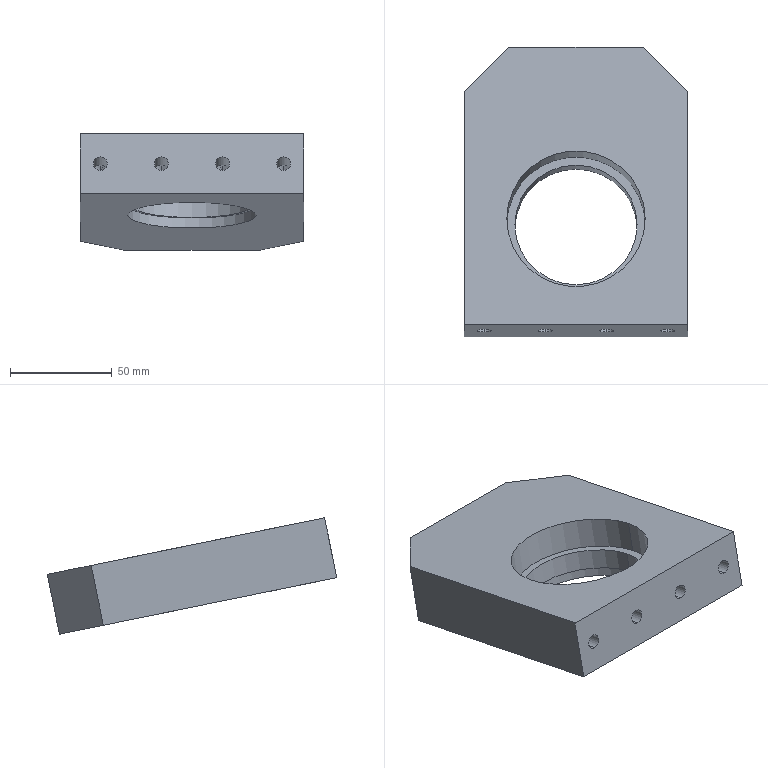Component | SolidWorks | JL001-04-01-004-2 | 1 solid | 32 faces | box 110 x 142.19 x 57.19 mm | volume 342876 mm3 | cylinder 14 | plane 10 | cone 8 | commonest cylinder face diameters 6.8 x8 63 x2 68 x2 60 x2
build123d program:
from build123d import *

# Parameters (mm, degrees)
SKETCH1_W             = 110
SKETCH1_H             = 139
BOSS_EXTRUDE1_DEPTH   = 15
SKETCH2_R             = 34
CUT_EXTRUDE1_DEPTH    = 15
SKETCH3_R             = 30
CUT_EXTRUDE2_DEPTH    = 90.89
M8_TAPPED_HOLE1_D     = 6.8
M8_TAPPED_HOLE1_DEPTH = 19.75
M8_TAPPED_HOLE1_TIP   = 2.043
SKETCH7_R             = 31.5
CUT_EXTRUDE3_DEPTH    = 5
CHAMFER1_SIZE         = 22


with BuildPart() as part:
    # Sketch1 → Boss-Extrude1 (new, symmetric)
    with BuildSketch(Plane.XY):
        Rectangle(SKETCH1_W, SKETCH1_H)
    extrude(amount=BOSS_EXTRUDE1_DEPTH, both=True)

    # Sketch2 → Cut-Extrude1 (cut)
    with BuildSketch(Plane.XY.offset(15)):
        with Locations((0, -16.5)):
            Circle(SKETCH2_R)
    extrude(amount=-CUT_EXTRUDE1_DEPTH, mode=Mode.SUBTRACT)

    # Sketch3 → Cut-Extrude2 (cut, through all)
    with BuildSketch(Plane.XY):
        with Locations((0, -16.5)):
            Circle(SKETCH3_R)
    extrude(amount=-CUT_EXTRUDE2_DEPTH, mode=Mode.SUBTRACT)

    # M8 Tapped Hole1
    with Locations(Plane(origin=(0, -69.5, 0), x_dir=(-1, 0, 0), z_dir=(0, -1, 0))):
        with Locations((45, 0), (15, 0), (-15, 0), (-45, 0)):
            Hole(M8_TAPPED_HOLE1_D / 2, depth=M8_TAPPED_HOLE1_DEPTH)
            with Locations((0, 0, -(M8_TAPPED_HOLE1_DEPTH + M8_TAPPED_HOLE1_TIP / 2))):  # 118° drill point
                Cone(0, M8_TAPPED_HOLE1_D / 2, M8_TAPPED_HOLE1_TIP, mode=Mode.SUBTRACT)

    # Sketch7 → Cut-Extrude3 (cut)
    with BuildSketch(Plane(origin=(0, 0, -15), x_dir=(-1, 0, 0), z_dir=(0, 0, -1))):
        with Locations((0, -16.5)):
            Circle(SKETCH7_R)
    extrude(amount=-CUT_EXTRUDE3_DEPTH, mode=Mode.SUBTRACT)

    # Chamfer1
    chamfer1_edges = [part.edges().sort_by_distance(p)[0] for p in [
        (-55, 69.5, 0),
        (55, 69.5, 0),
    ]]
    chamfer(chamfer1_edges, length=CHAMFER1_SIZE)


solid = part.part

# Placed as in the assembly
solid = solid.moved(Location((0, 185.894, -1.2), (-11.535, 0, 0)))
STEP:
#1=COLOUR_RGB('',0.7922,0.8196,0.9333);
#2=FILL_AREA_STYLE_COLOUR('',#1);
#3=FILL_AREA_STYLE('',(#2));
#4=SURFACE_STYLE_FILL_AREA(#3);
#5=SURFACE_SIDE_STYLE('',(#4));
#6=SURFACE_STYLE_USAGE(.BOTH.,#5);
#7=PRESENTATION_STYLE_ASSIGNMENT((#6));
#8=CARTESIAN_POINT('',(1.24,6.603,-0.3031));
#9=VERTEX_POINT('',#8);
#10=CARTESIAN_POINT('',(-1.24,6.603,-0.3031));
#11=VERTEX_POINT('',#10);
#12=CARTESIAN_POINT('',(-0.,6.603,-0.3031));
#13=DIRECTION('',(0.,-0.2,-0.9798));
#14=DIRECTION('',(-1.,0.,0.));
#15=AXIS2_PLACEMENT_3D('',#12,#13,#14);
#16=CIRCLE('',#15,1.24);
#17=EDGE_CURVE('',#9,#11,#16,.T.);
#18=ORIENTED_EDGE('',*,*,#17,.F.);
#19=CARTESIAN_POINT('',(1.24,6.564,-0.496));
#20=VERTEX_POINT('',#19);
#21=CARTESIAN_POINT('',(1.24,6.603,-0.3031));
#22=DIRECTION('',(0.,-0.2,-0.9798));
#23=VECTOR('',#22,39.37);
#24=LINE('',#21,#23);
#25=EDGE_CURVE('',#9,#20,#24,.T.);
#26=ORIENTED_EDGE('',*,*,#25,.T.);
#27=CARTESIAN_POINT('',(-1.24,6.564,-0.496));
#28=VERTEX_POINT('',#27);
#29=CARTESIAN_POINT('',(-0.,6.564,-0.496));
#30=DIRECTION('',(0.,-0.2,-0.9798));
#31=DIRECTION('',(-1.,0.,0.));
#32=AXIS2_PLACEMENT_3D('',#29,#30,#31);
#33=CIRCLE('',#32,1.24);
#34=EDGE_CURVE('',#20,#28,#33,.T.);
#35=ORIENTED_EDGE('',*,*,#34,.T.);
#36=CARTESIAN_POINT('',(-1.24,6.603,-0.3031));
#37=DIRECTION('',(0.,-0.2,-0.9798));
#38=VECTOR('',#37,39.37);
#39=LINE('',#36,#38);
#40=EDGE_CURVE('',#11,#28,#39,.T.);
#41=ORIENTED_EDGE('',*,*,#40,.F.);
#42=EDGE_LOOP('',(#18,#26,#35,#41));
#43=FACE_OUTER_BOUND('',#42,.T.);
#44=CARTESIAN_POINT('',(-0.,6.603,-0.3031));
#45=DIRECTION('',(0.,-0.2,-0.9798));
#46=DIRECTION('',(-1.,0.,0.));
#47=AXIS2_PLACEMENT_3D('',#44,#45,#46);
#48=CYLINDRICAL_SURFACE('',#47,1.24);
#49=ADVANCED_FACE('',(#43),#48,.F.);
#50=CARTESIAN_POINT('',(-1.772,5.426,0.4756));
#51=VERTEX_POINT('',#50);
#52=CARTESIAN_POINT('',(-1.772,5.373,0.2133));
#53=VERTEX_POINT('',#52);
#54=CARTESIAN_POINT('',(-1.772,5.4,0.3444));
#55=DIRECTION('',(-0.,-0.9798,0.2));
#56=DIRECTION('',(0.,-0.2,-0.9798));
#57=AXIS2_PLACEMENT_3D('',#54,#55,#56);
#58=CIRCLE('',#57,0.1339);
#59=EDGE_CURVE('',#51,#53,#58,.T.);
#60=ORIENTED_EDGE('',*,*,#59,.F.);
#61=CARTESIAN_POINT('',(-1.772,4.664,0.6311));
#62=VERTEX_POINT('',#61);
#63=CARTESIAN_POINT('',(-1.772,4.664,0.6311));
#64=DIRECTION('',(-0.,-0.9798,0.2));
#65=VECTOR('',#64,39.37);
#66=LINE('',#63,#65);
#67=EDGE_CURVE('',#51,#62,#66,.T.);
#68=ORIENTED_EDGE('',*,*,#67,.T.);
#69=CARTESIAN_POINT('',(-1.772,4.611,0.3687));
#70=VERTEX_POINT('',#69);
#71=CARTESIAN_POINT('',(-1.772,4.638,0.4999));
#72=DIRECTION('',(-0.,-0.9798,0.2));
#73=DIRECTION('',(0.,-0.2,-0.9798));
#74=AXIS2_PLACEMENT_3D('',#71,#72,#73);
#75=CIRCLE('',#74,0.1339);
#76=EDGE_CURVE('',#62,#70,#75,.T.);
#77=ORIENTED_EDGE('',*,*,#76,.T.);
#78=CARTESIAN_POINT('',(-1.772,4.611,0.3687));
#79=DIRECTION('',(-0.,-0.9798,0.2));
#80=VECTOR('',#79,39.37);
#81=LINE('',#78,#80);
#82=EDGE_CURVE('',#53,#70,#81,.T.);
#83=ORIENTED_EDGE('',*,*,#82,.F.);
#84=EDGE_LOOP('',(#60,#68,#77,#83));
#85=FACE_OUTER_BOUND('',#84,.T.);
#86=CARTESIAN_POINT('',(-1.772,4.638,0.4999));
#87=DIRECTION('',(-0.,-0.9798,0.2));
#88=DIRECTION('',(0.,-0.2,-0.9798));
#89=AXIS2_PLACEMENT_3D('',#86,#87,#88);
#90=CYLINDRICAL_SURFACE('',#89,0.1339);
#91=ADVANCED_FACE('',(#85),#90,.F.);
#92=CARTESIAN_POINT('',(-1.772,5.478,0.3283));
#93=VERTEX_POINT('',#92);
#94=CARTESIAN_POINT('',(-1.772,5.373,0.2133));
#95=DIRECTION('',(0.,-0.676,-0.7369));
#96=VECTOR('',#95,39.37);
#97=LINE('',#94,#96);
#98=EDGE_CURVE('',#93,#53,#97,.T.);
#99=ORIENTED_EDGE('',*,*,#98,.F.);
#100=CARTESIAN_POINT('',(-1.772,5.426,0.4756));
#101=DIRECTION('',(0.,-0.3332,0.9428));
#102=VECTOR('',#101,39.37);
#103=LINE('',#100,#102);
#104=EDGE_CURVE('',#93,#51,#103,.T.);
#105=ORIENTED_EDGE('',*,*,#104,.T.);
#106=ORIENTED_EDGE('',*,*,#59,.T.);
#107=EDGE_LOOP('',(#99,#105,#106));
#108=FACE_OUTER_BOUND('',#107,.T.);
#109=CARTESIAN_POINT('',(-1.772,5.4,0.3444));
#110=DIRECTION('',(-0.,-0.9798,0.2));
#111=DIRECTION('',(0.,-0.2,-0.9798));
#112=AXIS2_PLACEMENT_3D('',#109,#110,#111);
#113=CONICAL_SURFACE('',#112,0.1339,1.03);
#114=ADVANCED_FACE('',(#108),#113,.F.);
#115=CARTESIAN_POINT('',(-0.5906,5.426,0.4756));
#116=VERTEX_POINT('',#115);
#117=CARTESIAN_POINT('',(-0.5906,5.373,0.2133));
#118=VERTEX_POINT('',#117);
#119=CARTESIAN_POINT('',(-0.5906,5.4,0.3444));
#120=DIRECTION('',(-0.,-0.9798,0.2));
#121=DIRECTION('',(0.,-0.2,-0.9798));
#122=AXIS2_PLACEMENT_3D('',#119,#120,#121);
#123=CIRCLE('',#122,0.1339);
#124=EDGE_CURVE('',#116,#118,#123,.T.);
#125=ORIENTED_EDGE('',*,*,#124,.F.);
#126=CARTESIAN_POINT('',(-0.5906,4.664,0.6311));
#127=VERTEX_POINT('',#126);
#128=CARTESIAN_POINT('',(-0.5906,4.664,0.6311));
#129=DIRECTION('',(-0.,-0.9798,0.2));
#130=VECTOR('',#129,39.37);
#131=LINE('',#128,#130);
#132=EDGE_CURVE('',#116,#127,#131,.T.);
#133=ORIENTED_EDGE('',*,*,#132,.T.);
#134=CARTESIAN_POINT('',(-0.5906,4.611,0.3687));
#135=VERTEX_POINT('',#134);
#136=CARTESIAN_POINT('',(-0.5906,4.638,0.4999));
#137=DIRECTION('',(-0.,-0.9798,0.2));
#138=DIRECTION('',(0.,-0.2,-0.9798));
#139=AXIS2_PLACEMENT_3D('',#136,#137,#138);
#140=CIRCLE('',#139,0.1339);
#141=EDGE_CURVE('',#127,#135,#140,.T.);
#142=ORIENTED_EDGE('',*,*,#141,.T.);
#143=CARTESIAN_POINT('',(-0.5906,4.611,0.3687));
#144=DIRECTION('',(-0.,-0.9798,0.2));
#145=VECTOR('',#144,39.37);
#146=LINE('',#143,#145);
#147=EDGE_CURVE('',#118,#135,#146,.T.);
#148=ORIENTED_EDGE('',*,*,#147,.F.);
#149=EDGE_LOOP('',(#125,#133,#142,#148));
#150=FACE_OUTER_BOUND('',#149,.T.);
#151=CARTESIAN_POINT('',(-0.5906,4.638,0.4999));
#152=DIRECTION('',(-0.,-0.9798,0.2));
#153=DIRECTION('',(0.,-0.2,-0.9798));
#154=AXIS2_PLACEMENT_3D('',#151,#152,#153);
#155=CYLINDRICAL_SURFACE('',#154,0.1339);
#156=ADVANCED_FACE('',(#150),#155,.F.);
#157=CARTESIAN_POINT('',(-0.5906,5.478,0.3283));
#158=VERTEX_POINT('',#157);
#159=CARTESIAN_POINT('',(-0.5906,5.373,0.2133));
#160=DIRECTION('',(0.,-0.676,-0.7369));
#161=VECTOR('',#160,39.37);
#162=LINE('',#159,#161);
#163=EDGE_CURVE('',#158,#118,#162,.T.);
#164=ORIENTED_EDGE('',*,*,#163,.F.);
#165=CARTESIAN_POINT('',(-0.5906,5.426,0.4756));
#166=DIRECTION('',(0.,-0.3332,0.9428));
#167=VECTOR('',#166,39.37);
#168=LINE('',#165,#167);
#169=EDGE_CURVE('',#158,#116,#168,.T.);
#170=ORIENTED_EDGE('',*,*,#169,.T.);
#171=ORIENTED_EDGE('',*,*,#124,.T.);
#172=EDGE_LOOP('',(#164,#170,#171));
#173=FACE_OUTER_BOUND('',#172,.T.);
#174=CARTESIAN_POINT('',(-0.5906,5.4,0.3444));
#175=DIRECTION('',(-0.,-0.9798,0.2));
#176=DIRECTION('',(0.,-0.2,-0.9798));
#177=AXIS2_PLACEMENT_3D('',#174,#175,#176);
#178=CONICAL_SURFACE('',#177,0.1339,1.03);
#179=ADVANCED_FACE('',(#173),#178,.F.);
#180=CARTESIAN_POINT('',(0.5906,5.426,0.4756));
#181=VERTEX_POINT('',#180);
#182=CARTESIAN_POINT('',(0.5906,5.373,0.2133));
#183=VERTEX_POINT('',#182);
#184=CARTESIAN_POINT('',(0.5906,5.4,0.3444));
#185=DIRECTION('',(-0.,-0.9798,0.2));
#186=DIRECTION('',(0.,-0.2,-0.9798));
#187=AXIS2_PLACEMENT_3D('',#184,#185,#186);
#188=CIRCLE('',#187,0.1339);
#189=EDGE_CURVE('',#181,#183,#188,.T.);
#190=ORIENTED_EDGE('',*,*,#189,.F.);
#191=CARTESIAN_POINT('',(0.5906,4.664,0.6311));
#192=VERTEX_POINT('',#191);
#193=CARTESIAN_POINT('',(0.5906,4.664,0.6311));
#194=DIRECTION('',(-0.,-0.9798,0.2));
#195=VECTOR('',#194,39.37);
#196=LINE('',#193,#195);
#197=EDGE_CURVE('',#181,#192,#196,.T.);
#198=ORIENTED_EDGE('',*,*,#197,.T.);
#199=CARTESIAN_POINT('',(0.5906,4.611,0.3687));
#200=VERTEX_POINT('',#199);
#201=CARTESIAN_POINT('',(0.5906,4.638,0.4999));
#202=DIRECTION('',(-0.,-0.9798,0.2));
#203=DIRECTION('',(0.,-0.2,-0.9798));
#204=AXIS2_PLACEMENT_3D('',#201,#202,#203);
#205=CIRCLE('',#204,0.1339);
#206=EDGE_CURVE('',#192,#200,#205,.T.);
#207=ORIENTED_EDGE('',*,*,#206,.T.);
#208=CARTESIAN_POINT('',(0.5906,4.611,0.3687));
#209=DIRECTION('',(-0.,-0.9798,0.2));
#210=VECTOR('',#209,39.37);
#211=LINE('',#208,#210);
#212=EDGE_CURVE('',#183,#200,#211,.T.);
#213=ORIENTED_EDGE('',*,*,#212,.F.);
#214=EDGE_LOOP('',(#190,#198,#207,#213));
#215=FACE_OUTER_BOUND('',#214,.T.);
#216=CARTESIAN_POINT('',(0.5906,4.638,0.4999));
#217=DIRECTION('',(-0.,-0.9798,0.2));
#218=DIRECTION('',(0.,-0.2,-0.9798));
#219=AXIS2_PLACEMENT_3D('',#216,#217,#218);
#220=CYLINDRICAL_SURFACE('',#219,0.1339);
#221=ADVANCED_FACE('',(#215),#220,.F.);
#222=CARTESIAN_POINT('',(0.5906,5.478,0.3283));
#223=VERTEX_POINT('',#222);
#224=CARTESIAN_POINT('',(0.5906,5.373,0.2133));
#225=DIRECTION('',(0.,-0.676,-0.7369));
#226=VECTOR('',#225,39.37);
#227=LINE('',#224,#226);
#228=EDGE_CURVE('',#223,#183,#227,.T.);
#229=ORIENTED_EDGE('',*,*,#228,.F.);
#230=CARTESIAN_POINT('',(0.5906,5.426,0.4756));
#231=DIRECTION('',(0.,-0.3332,0.9428));
#232=VECTOR('',#231,39.37);
#233=LINE('',#230,#232);
#234=EDGE_CURVE('',#223,#181,#233,.T.);
#235=ORIENTED_EDGE('',*,*,#234,.T.);
#236=ORIENTED_EDGE('',*,*,#189,.T.);
#237=EDGE_LOOP('',(#229,#235,#236));
#238=FACE_OUTER_BOUND('',#237,.T.);
#239=CARTESIAN_POINT('',(0.5906,5.4,0.3444));
#240=DIRECTION('',(-0.,-0.9798,0.2));
#241=DIRECTION('',(0.,-0.2,-0.9798));
#242=AXIS2_PLACEMENT_3D('',#239,#240,#241);
#243=CONICAL_SURFACE('',#242,0.1339,1.03);
#244=ADVANCED_FACE('',(#238),#243,.F.);
#245=CARTESIAN_POINT('',(1.772,5.426,0.4756));
#246=VERTEX_POINT('',#245);
#247=CARTESIAN_POINT('',(1.772,5.373,0.2133));
#248=VERTEX_POINT('',#247);
#249=CARTESIAN_POINT('',(1.772,5.4,0.3444));
#250=DIRECTION('',(-0.,-0.9798,0.2));
#251=DIRECTION('',(0.,-0.2,-0.9798));
#252=AXIS2_PLACEMENT_3D('',#249,#250,#251);
#253=CIRCLE('',#252,0.1339);
#254=EDGE_CURVE('',#246,#248,#253,.T.);
#255=ORIENTED_EDGE('',*,*,#254,.F.);
#256=CARTESIAN_POINT('',(1.772,4.664,0.6311));
#257=VERTEX_POINT('',#256);
#258=CARTESIAN_POINT('',(1.772,4.664,0.6311));
#259=DIRECTION('',(-0.,-0.9798,0.2));
#260=VECTOR('',#259,39.37);
#261=LINE('',#258,#260);
#262=EDGE_CURVE('',#246,#257,#261,.T.);
#263=ORIENTED_EDGE('',*,*,#262,.T.);
#264=CARTESIAN_POINT('',(1.772,4.611,0.3687));
#265=VERTEX_POINT('',#264);
#266=CARTESIAN_POINT('',(1.772,4.638,0.4999));
#267=DIRECTION('',(-0.,-0.9798,0.2));
#268=DIRECTION('',(0.,-0.2,-0.9798));
#269=AXIS2_PLACEMENT_3D('',#266,#267,#268);
#270=CIRCLE('',#269,0.1339);
#271=EDGE_CURVE('',#257,#265,#270,.T.);
#272=ORIENTED_EDGE('',*,*,#271,.T.);
#273=CARTESIAN_POINT('',(1.772,4.611,0.3687));
#274=DIRECTION('',(-0.,-0.9798,0.2));
#275=VECTOR('',#274,39.37);
#276=LINE('',#273,#275);
#277=EDGE_CURVE('',#248,#265,#276,.T.);
#278=ORIENTED_EDGE('',*,*,#277,.F.);
#279=EDGE_LOOP('',(#255,#263,#272,#278));
#280=FACE_OUTER_BOUND('',#279,.T.);
#281=CARTESIAN_POINT('',(1.772,4.638,0.4999));
#282=DIRECTION('',(-0.,-0.9798,0.2));
#283=DIRECTION('',(0.,-0.2,-0.9798));
#284=AXIS2_PLACEMENT_3D('',#281,#282,#283);
#285=CYLINDRICAL_SURFACE('',#284,0.1339);
#286=ADVANCED_FACE('',(#280),#285,.F.);
#287=CARTESIAN_POINT('',(1.772,5.478,0.3283));
#288=VERTEX_POINT('',#287);
#289=CARTESIAN_POINT('',(1.772,5.373,0.2133));
#290=DIRECTION('',(0.,-0.676,-0.7369));
#291=VECTOR('',#290,39.37);
#292=LINE('',#289,#291);
#293=EDGE_CURVE('',#288,#248,#292,.T.);
#294=ORIENTED_EDGE('',*,*,#293,.F.);
#295=CARTESIAN_POINT('',(1.772,5.426,0.4756));
#296=DIRECTION('',(0.,-0.3332,0.9428));
#297=VECTOR('',#296,39.37);
#298=LINE('',#295,#297);
#299=EDGE_CURVE('',#288,#246,#298,.T.);
#300=ORIENTED_EDGE('',*,*,#299,.T.);
#301=ORIENTED_EDGE('',*,*,#254,.T.);
#302=EDGE_LOOP('',(#294,#300,#301));
#303=FACE_OUTER_BOUND('',#302,.T.);
#304=CARTESIAN_POINT('',(1.772,5.4,0.3444));
#305=DIRECTION('',(-0.,-0.9798,0.2));
#306=DIRECTION('',(0.,-0.2,-0.9798));
#307=AXIS2_PLACEMENT_3D('',#304,#305,#306);
#308=CONICAL_SURFACE('',#307,0.1339,1.03);
#309=ADVANCED_FACE('',(#303),#308,.F.);
#310=CARTESIAN_POINT('',(-1.339,6.682,0.08266));
#311=VERTEX_POINT('',#310);
#312=CARTESIAN_POINT('',(1.339,6.682,0.08266));
#313=VERTEX_POINT('',#312);
#314=CARTESIAN_POINT('',(-0.,6.682,0.08266));
#315=DIRECTION('',(-0.,0.2,0.9798));
#316=DIRECTION('',(1.,0.,0.));
#317=AXIS2_PLACEMENT_3D('',#314,#315,#316);
#318=CIRCLE('',#317,1.339);
#319=EDGE_CURVE('',#311,#313,#318,.T.);
#320=ORIENTED_EDGE('',*,*,#319,.F.);
#321=CARTESIAN_POINT('',(-1.339,6.8,0.6613));
#322=VERTEX_POINT('',#321);
#323=CARTESIAN_POINT('',(-1.339,6.682,0.08266));
#324=DIRECTION('',(-0.,0.2,0.9798));
#325=VECTOR('',#324,39.37);
#326=LINE('',#323,#325);
#327=EDGE_CURVE('',#311,#322,#326,.T.);
#328=ORIENTED_EDGE('',*,*,#327,.T.);
#329=CARTESIAN_POINT('',(1.339,6.8,0.6613));
#330=VERTEX_POINT('',#329);
#331=CARTESIAN_POINT('',(-0.,6.8,0.6613));
#332=DIRECTION('',(-0.,0.2,0.9798));
#333=DIRECTION('',(1.,0.,0.));
#334=AXIS2_PLACEMENT_3D('',#331,#332,#333);
#335=CIRCLE('',#334,1.339);
#336=EDGE_CURVE('',#322,#330,#335,.T.);
#337=ORIENTED_EDGE('',*,*,#336,.T.);
#338=CARTESIAN_POINT('',(1.339,6.682,0.08266));
#339=DIRECTION('',(-0.,0.2,0.9798));
#340=VECTOR('',#339,39.37);
#341=LINE('',#338,#340);
#342=EDGE_CURVE('',#313,#330,#341,.T.);
#343=ORIENTED_EDGE('',*,*,#342,.F.);
#344=EDGE_LOOP('',(#320,#328,#337,#343));
#345=FACE_OUTER_BOUND('',#344,.T.);
#346=CARTESIAN_POINT('',(-0.,6.682,0.08266));
#347=DIRECTION('',(-0.,0.2,0.9798));
#348=DIRECTION('',(1.,0.,0.));
#349=AXIS2_PLACEMENT_3D('',#346,#347,#348);
#350=CYLINDRICAL_SURFACE('',#349,1.339);
#351=ADVANCED_FACE('',(#345),#350,.F.);
#352=CARTESIAN_POINT('',(-1.181,6.603,-0.3031));
#353=VERTEX_POINT('',#352);
#354=CARTESIAN_POINT('',(1.181,6.603,-0.3031));
#355=VERTEX_POINT('',#354);
#356=CARTESIAN_POINT('',(-0.,6.603,-0.3031));
#357=DIRECTION('',(-0.,0.2,0.9798));
#358=DIRECTION('',(-1.,0.,0.));
#359=AXIS2_PLACEMENT_3D('',#356,#357,#358);
#360=CIRCLE('',#359,1.181);
#361=EDGE_CURVE('',#353,#355,#360,.T.);
#362=ORIENTED_EDGE('',*,*,#361,.F.);
#363=CARTESIAN_POINT('',(-1.181,6.682,0.08266));
#364=VERTEX_POINT('',#363);
#365=CARTESIAN_POINT('',(-1.181,6.564,-0.496));
#366=DIRECTION('',(-0.,0.2,0.9798));
#367=VECTOR('',#366,39.37);
#368=LINE('',#365,#367);
#369=EDGE_CURVE('',#353,#364,#368,.T.);
#370=ORIENTED_EDGE('',*,*,#369,.T.);
#371=CARTESIAN_POINT('',(1.181,6.682,0.08266));
#372=VERTEX_POINT('',#371);
#373=CARTESIAN_POINT('',(-0.,6.682,0.08266));
#374=DIRECTION('',(-0.,0.2,0.9798));
#375=DIRECTION('',(1.,0.,0.));
#376=AXIS2_PLACEMENT_3D('',#373,#374,#375);
#377=CIRCLE('',#376,1.181);
#378=EDGE_CURVE('',#364,#372,#377,.T.);
#379=ORIENTED_EDGE('',*,*,#378,.T.);
#380=CARTESIAN_POINT('',(1.181,6.564,-0.496));
#381=DIRECTION('',(-0.,0.2,0.9798));
#382=VECTOR('',#381,39.37);
#383=LINE('',#380,#382);
#384=EDGE_CURVE('',#355,#372,#383,.T.);
#385=ORIENTED_EDGE('',*,*,#384,.F.);
#386=EDGE_LOOP('',(#362,#370,#379,#385));
#387=FACE_OUTER_BOUND('',#386,.T.);
#388=CARTESIAN_POINT('',(-0.,6.564,-0.496));
#389=DIRECTION('',(-0.,0.2,0.9798));
#390=DIRECTION('',(1.,0.,0.));
#391=AXIS2_PLACEMENT_3D('',#388,#389,#390);
#392=CYLINDRICAL_SURFACE('',#391,1.181);
#393=ADVANCED_FACE('',(#387),#392,.F.);
#394=ORIENTED_EDGE('',*,*,#369,.F.);
#395=CARTESIAN_POINT('',(-0.,6.603,-0.3031));
#396=DIRECTION('',(-0.,0.2,0.9798));
#397=DIRECTION('',(-1.,0.,0.));
#398=AXIS2_PLACEMENT_3D('',#395,#396,#397);
#399=CIRCLE('',#398,1.181);
#400=EDGE_CURVE('',#355,#353,#399,.T.);
#401=ORIENTED_EDGE('',*,*,#400,.F.);
#402=ORIENTED_EDGE('',*,*,#384,.T.);
#403=CARTESIAN_POINT('',(-0.,6.682,0.08266));
#404=DIRECTION('',(-0.,0.2,0.9798));
#405=DIRECTION('',(1.,0.,0.));
#406=AXIS2_PLACEMENT_3D('',#403,#404,#405);
#407=CIRCLE('',#406,1.181);
#408=EDGE_CURVE('',#372,#364,#407,.T.);
#409=ORIENTED_EDGE('',*,*,#408,.T.);
#410=EDGE_LOOP('',(#394,#401,#402,#409));
#411=FACE_OUTER_BOUND('',#410,.T.);
#412=CARTESIAN_POINT('',(-0.,6.564,-0.496));
#413=DIRECTION('',(-0.,0.2,0.9798));
#414=DIRECTION('',(1.,0.,0.));
#415=AXIS2_PLACEMENT_3D('',#412,#413,#414);
#416=CYLINDRICAL_SURFACE('',#415,1.181);
#417=ADVANCED_FACE('',(#411),#416,.F.);
#418=CARTESIAN_POINT('',(2.165,4.52,-0.07872));
#419=VERTEX_POINT('',#418);
#420=CARTESIAN_POINT('',(2.165,9.033,-0.9998));
#421=VERTEX_POINT('',#420);
#422=CARTESIAN_POINT('',(2.165,9.882,-1.173));
#423=DIRECTION('',(0.,0.9798,-0.2));
#424=VECTOR('',#423,39.37);
#425=LINE('',#422,#424);
#426=EDGE_CURVE('',#419,#421,#425,.T.);
#427=ORIENTED_EDGE('',*,*,#426,.T.);
#428=CARTESIAN_POINT('',(2.165,9.269,0.1574));
#429=VERTEX_POINT('',#428);
#430=CARTESIAN_POINT('',(2.165,9.269,0.1574));
#431=DIRECTION('',(-0.,0.2,0.9798));
#432=VECTOR('',#431,39.37);
#433=LINE('',#430,#432);
#434=EDGE_CURVE('',#421,#429,#433,.T.);
#435=ORIENTED_EDGE('',*,*,#434,.T.);
#436=CARTESIAN_POINT('',(2.165,4.756,1.079));
#437=VERTEX_POINT('',#436);
#438=CARTESIAN_POINT('',(2.165,10.118,-0.01574));
#439=DIRECTION('',(0.,0.9798,-0.2));
#440=VECTOR('',#439,39.37);
#441=LINE('',#438,#440);
#442=EDGE_CURVE('',#437,#429,#441,.T.);
#443=ORIENTED_EDGE('',*,*,#442,.F.);
#444=CARTESIAN_POINT('',(2.165,4.756,1.079));
#445=DIRECTION('',(0.,-0.2,-0.9798));
#446=VECTOR('',#445,39.37);
#447=LINE('',#444,#446);
#448=EDGE_CURVE('',#437,#419,#447,.T.);
#449=ORIENTED_EDGE('',*,*,#448,.T.);
#450=EDGE_LOOP('',(#427,#435,#443,#449));
#451=FACE_OUTER_BOUND('',#450,.T.);
#452=CARTESIAN_POINT('',(2.165,10.118,-0.01574));
#453=DIRECTION('',(-1.,-0.,-0.));
#454=DIRECTION('',(-0.,0.2,0.9798));
#455=AXIS2_PLACEMENT_3D('',#452,#453,#454);
#456=PLANE('',#455);
#457=ADVANCED_FACE('',(#451),#456,.F.);
#458=CARTESIAN_POINT('',(1.299,9.882,-1.173));
#459=VERTEX_POINT('',#458);
#460=CARTESIAN_POINT('',(-1.299,9.882,-1.173));
#461=VERTEX_POINT('',#460);
#462=CARTESIAN_POINT('',(-2.165,9.882,-1.173));
#463=DIRECTION('',(-1.,-0.,-0.));
#464=VECTOR('',#463,39.37);
#465=LINE('',#462,#464);
#466=EDGE_CURVE('',#459,#461,#465,.T.);
#467=ORIENTED_EDGE('',*,*,#466,.T.);
#468=CARTESIAN_POINT('',(-1.299,10.118,-0.01574));
#469=VERTEX_POINT('',#468);
#470=CARTESIAN_POINT('',(-1.299,10.118,-0.01574));
#471=DIRECTION('',(-0.,0.2,0.9798));
#472=VECTOR('',#471,39.37);
#473=LINE('',#470,#472);
#474=EDGE_CURVE('',#461,#469,#473,.T.);
#475=ORIENTED_EDGE('',*,*,#474,.T.);
#476=CARTESIAN_POINT('',(1.299,10.118,-0.01574));
#477=VERTEX_POINT('',#476);
#478=CARTESIAN_POINT('',(-2.165,10.118,-0.01574));
#479=DIRECTION('',(-1.,-0.,-0.));
#480=VECTOR('',#479,39.37);
#481=LINE('',#478,#480);
#482=EDGE_CURVE('',#477,#469,#481,.T.);
#483=ORIENTED_EDGE('',*,*,#482,.F.);
#484=CARTESIAN_POINT('',(1.299,10.118,-0.01574));
#485=DIRECTION('',(0.,-0.2,-0.9798));
#486=VECTOR('',#485,39.37);
#487=LINE('',#484,#486);
#488=EDGE_CURVE('',#477,#459,#487,.T.);
#489=ORIENTED_EDGE('',*,*,#488,.T.);
#490=EDGE_LOOP('',(#467,#475,#483,#489));
#491=FACE_OUTER_BOUND('',#490,.T.);
#492=CARTESIAN_POINT('',(-2.165,10.118,-0.01574));
#493=DIRECTION('',(-0.,-0.9798,0.2));
#494=DIRECTION('',(0.,-0.2,-0.9798));
#495=AXIS2_PLACEMENT_3D('',#492,#493,#494);
#496=PLANE('',#495);
#497=ADVANCED_FACE('',(#491),#496,.F.);
#498=CARTESIAN_POINT('',(-2.165,9.269,0.1574));
#499=VERTEX_POINT('',#498);
#500=CARTESIAN_POINT('',(-2.165,4.756,1.079));
#501=VERTEX_POINT('',#500);
#502=CARTESIAN_POINT('',(-2.165,10.118,-0.01574));
#503=DIRECTION('',(0.,-0.9798,0.2));
#504=VECTOR('',#503,39.37);
#505=LINE('',#502,#504);
#506=EDGE_CURVE('',#499,#501,#505,.T.);
#507=ORIENTED_EDGE('',*,*,#506,.F.);
#508=CARTESIAN_POINT('',(-2.165,9.033,-0.9998));
#509=VERTEX_POINT('',#508);
#510=CARTESIAN_POINT('',(-2.165,9.269,0.1574));
#511=DIRECTION('',(0.,-0.2,-0.9798));
#512=VECTOR('',#511,39.37);
#513=LINE('',#510,#512);
#514=EDGE_CURVE('',#499,#509,#513,.T.);
#515=ORIENTED_EDGE('',*,*,#514,.T.);
#516=CARTESIAN_POINT('',(-2.165,4.52,-0.07872));
#517=VERTEX_POINT('',#516);
#518=CARTESIAN_POINT('',(-2.165,9.882,-1.173));
#519=DIRECTION('',(0.,-0.9798,0.2));
#520=VECTOR('',#519,39.37);
#521=LINE('',#518,#520);
#522=EDGE_CURVE('',#509,#517,#521,.T.);
#523=ORIENTED_EDGE('',*,*,#522,.T.);
#524=CARTESIAN_POINT('',(-2.165,4.756,1.079));
#525=DIRECTION('',(0.,-0.2,-0.9798));
#526=VECTOR('',#525,39.37);
#527=LINE('',#524,#526);
#528=EDGE_CURVE('',#501,#517,#527,.T.);
#529=ORIENTED_EDGE('',*,*,#528,.F.);
#530=EDGE_LOOP('',(#507,#515,#523,#529));
#531=FACE_OUTER_BOUND('',#530,.T.);
#532=CARTESIAN_POINT('',(-2.165,10.118,-0.01574));
#533=DIRECTION('',(1.,0.,-0.));
#534=DIRECTION('',(-0.,0.9798,-0.2));
#535=AXIS2_PLACEMENT_3D('',#532,#533,#534);
#536=PLANE('',#535);
#537=ADVANCED_FACE('',(#531),#536,.F.);
#538=CARTESIAN_POINT('',(-1.772,4.638,0.4999));
#539=DIRECTION('',(-0.,-0.9798,0.2));
#540=DIRECTION('',(0.,-0.2,-0.9798));
#541=AXIS2_PLACEMENT_3D('',#538,#539,#540);
#542=CIRCLE('',#541,0.1339);
#543=EDGE_CURVE('',#70,#62,#542,.T.);
#544=ORIENTED_EDGE('',*,*,#543,.F.);
#545=ORIENTED_EDGE('',*,*,#76,.F.);
#546=EDGE_LOOP('',(#544,#545));
#547=FACE_BOUND('',#546,.T.);
#548=CARTESIAN_POINT('',(-0.5906,4.638,0.4999));
#549=DIRECTION('',(-0.,-0.9798,0.2));
#550=DIRECTION('',(0.,-0.2,-0.9798));
#551=AXIS2_PLACEMENT_3D('',#548,#549,#550);
#552=CIRCLE('',#551,0.1339);
#553=EDGE_CURVE('',#135,#127,#552,.T.);
#554=ORIENTED_EDGE('',*,*,#553,.F.);
#555=ORIENTED_EDGE('',*,*,#141,.F.);
#556=EDGE_LOOP('',(#554,#555));
#557=FACE_BOUND('',#556,.T.);
#558=CARTESIAN_POINT('',(0.5906,4.638,0.4999));
#559=DIRECTION('',(-0.,-0.9798,0.2));
#560=DIRECTION('',(0.,-0.2,-0.9798));
#561=AXIS2_PLACEMENT_3D('',#558,#559,#560);
#562=CIRCLE('',#561,0.1339);
#563=EDGE_CURVE('',#200,#192,#562,.T.);
#564=ORIENTED_EDGE('',*,*,#563,.F.);
#565=ORIENTED_EDGE('',*,*,#206,.F.);
#566=EDGE_LOOP('',(#564,#565));
#567=FACE_BOUND('',#566,.T.);
#568=CARTESIAN_POINT('',(1.772,4.638,0.4999));
#569=DIRECTION('',(-0.,-0.9798,0.2));
#570=DIRECTION('',(0.,-0.2,-0.9798));
#571=AXIS2_PLACEMENT_3D('',#568,#569,#570);
#572=CIRCLE('',#571,0.1339);
#573=EDGE_CURVE('',#265,#257,#572,.T.);
#574=ORIENTED_EDGE('',*,*,#573,.F.);
#575=ORIENTED_EDGE('',*,*,#271,.F.);
#576=EDGE_LOOP('',(#574,#575));
#577=FACE_BOUND('',#576,.T.);
#578=CARTESIAN_POINT('',(-2.165,4.52,-0.07872));
#579=DIRECTION('',(1.,0.,0.));
#580=VECTOR('',#579,39.37);
#581=LINE('',#578,#580);
#582=EDGE_CURVE('',#517,#419,#581,.T.);
#583=ORIENTED_EDGE('',*,*,#582,.T.);
#584=ORIENTED_EDGE('',*,*,#448,.F.);
#585=CARTESIAN_POINT('',(-2.165,4.756,1.079));
#586=DIRECTION('',(1.,0.,0.));
#587=VECTOR('',#586,39.37);
#588=LINE('',#585,#587);
#589=EDGE_CURVE('',#501,#437,#588,.T.);
#590=ORIENTED_EDGE('',*,*,#589,.F.);
#591=ORIENTED_EDGE('',*,*,#528,.T.);
#592=EDGE_LOOP('',(#583,#584,#590,#591));
#593=FACE_OUTER_BOUND('',#592,.T.);
#594=CARTESIAN_POINT('',(-2.165,4.756,1.079));
#595=DIRECTION('',(0.,0.9798,-0.2));
#596=DIRECTION('',(-0.,0.2,0.9798));
#597=AXIS2_PLACEMENT_3D('',#594,#595,#596);
#598=PLANE('',#597);
#599=ADVANCED_FACE('',(#547,#557,#567,#577,#593),#598,.F.);
#600=CARTESIAN_POINT('',(-0.,6.8,0.6613));
#601=DIRECTION('',(-0.,0.2,0.9798));
#602=DIRECTION('',(1.,0.,0.));
#603=AXIS2_PLACEMENT_3D('',#600,#601,#602);
#604=CIRCLE('',#603,1.339);
#605=EDGE_CURVE('',#330,#322,#604,.T.);
#606=ORIENTED_EDGE('',*,*,#605,.F.);
#607=ORIENTED_EDGE('',*,*,#336,.F.);
#608=EDGE_LOOP('',(#606,#607));
#609=FACE_BOUND('',#608,.T.);
#610=ORIENTED_EDGE('',*,*,#482,.T.);
#611=CARTESIAN_POINT('',(-2.018,9.414,0.1279));
#612=DIRECTION('',(-0.7071,-0.6928,0.1414));
#613=VECTOR('',#612,39.37);
#614=LINE('',#611,#613);
#615=EDGE_CURVE('',#469,#499,#614,.T.);
#616=ORIENTED_EDGE('',*,*,#615,.T.);
#617=ORIENTED_EDGE('',*,*,#506,.T.);
#618=ORIENTED_EDGE('',*,*,#589,.T.);
#619=ORIENTED_EDGE('',*,*,#442,.T.);
#620=CARTESIAN_POINT('',(2.018,9.414,0.1279));
#621=DIRECTION('',(-0.7071,0.6928,-0.1414));
#622=VECTOR('',#621,39.37);
#623=LINE('',#620,#622);
#624=EDGE_CURVE('',#429,#477,#623,.T.);
#625=ORIENTED_EDGE('',*,*,#624,.T.);
#626=EDGE_LOOP('',(#610,#616,#617,#618,#619,#625));
#627=FACE_OUTER_BOUND('',#626,.T.);
#628=CARTESIAN_POINT('',(-0.,7.437,0.5314));
#629=DIRECTION('',(-0.,0.2,0.9798));
#630=DIRECTION('',(1.,0.,0.));
#631=AXIS2_PLACEMENT_3D('',#628,#629,#630);
#632=PLANE('',#631);
#633=ADVANCED_FACE('',(#609,#627),#632,.T.);
#634=CARTESIAN_POINT('',(-0.,6.564,-0.496));
#635=DIRECTION('',(0.,-0.2,-0.9798));
#636=DIRECTION('',(-1.,0.,0.));
#637=AXIS2_PLACEMENT_3D('',#634,#635,#636);
#638=CIRCLE('',#637,1.24);
#639=EDGE_CURVE('',#28,#20,#638,.T.);
#640=ORIENTED_EDGE('',*,*,#639,.F.);
#641=ORIENTED_EDGE('',*,*,#34,.F.);
#642=EDGE_LOOP('',(#640,#641));
#643=FACE_BOUND('',#642,.T.);
#644=ORIENTED_EDGE('',*,*,#522,.F.);
#645=CARTESIAN_POINT('',(-2.165,9.033,-0.9998));
#646=DIRECTION('',(0.7071,0.6928,-0.1414));
#647=VECTOR('',#646,39.37);
#648=LINE('',#645,#647);
#649=EDGE_CURVE('',#509,#461,#648,.T.);
#650=ORIENTED_EDGE('',*,*,#649,.T.);
#651=ORIENTED_EDGE('',*,*,#466,.F.);
#652=CARTESIAN_POINT('',(1.299,9.882,-1.173));
#653=DIRECTION('',(0.7071,-0.6928,0.1414));
#654=VECTOR('',#653,39.37);
#655=LINE('',#652,#654);
#656=EDGE_CURVE('',#459,#421,#655,.T.);
#657=ORIENTED_EDGE('',*,*,#656,.T.);
#658=ORIENTED_EDGE('',*,*,#426,.F.);
#659=ORIENTED_EDGE('',*,*,#582,.F.);
#660=EDGE_LOOP('',(#644,#650,#651,#657,#658,#659));
#661=FACE_OUTER_BOUND('',#660,.T.);
#662=CARTESIAN_POINT('',(-0.,7.201,-0.6259));
#663=DIRECTION('',(-0.,0.2,0.9798));
#664=DIRECTION('',(1.,0.,0.));
#665=AXIS2_PLACEMENT_3D('',#662,#663,#664);
#666=PLANE('',#665);
#667=ADVANCED_FACE('',(#643,#661),#666,.F.);
#668=ORIENTED_EDGE('',*,*,#327,.F.);
#669=CARTESIAN_POINT('',(-0.,6.682,0.08266));
#670=DIRECTION('',(-0.,0.2,0.9798));
#671=DIRECTION('',(1.,0.,0.));
#672=AXIS2_PLACEMENT_3D('',#669,#670,#671);
#673=CIRCLE('',#672,1.339);
#674=EDGE_CURVE('',#313,#311,#673,.T.);
#675=ORIENTED_EDGE('',*,*,#674,.F.);
#676=ORIENTED_EDGE('',*,*,#342,.T.);
#677=ORIENTED_EDGE('',*,*,#605,.T.);
#678=EDGE_LOOP('',(#668,#675,#676,#677));
#679=FACE_OUTER_BOUND('',#678,.T.);
#680=CARTESIAN_POINT('',(-0.,6.682,0.08266));
#681=DIRECTION('',(-0.,0.2,0.9798));
#682=DIRECTION('',(1.,0.,0.));
#683=AXIS2_PLACEMENT_3D('',#680,#681,#682);
#684=CYLINDRICAL_SURFACE('',#683,1.339);
#685=ADVANCED_FACE('',(#679),#684,.F.);
#686=ORIENTED_EDGE('',*,*,#408,.F.);
#687=ORIENTED_EDGE('',*,*,#378,.F.);
#688=EDGE_LOOP('',(#686,#687));
#689=FACE_BOUND('',#688,.T.);
#690=ORIENTED_EDGE('',*,*,#674,.T.);
#691=ORIENTED_EDGE('',*,*,#319,.T.);
#692=EDGE_LOOP('',(#690,#691));
#693=FACE_OUTER_BOUND('',#692,.T.);
#694=CARTESIAN_POINT('',(-0.,6.682,0.08266));
#695=DIRECTION('',(-0.,0.2,0.9798));
#696=DIRECTION('',(1.,0.,0.));
#697=AXIS2_PLACEMENT_3D('',#694,#695,#696);
#698=PLANE('',#697);
#699=ADVANCED_FACE('',(#689,#693),#698,.T.);
#700=ORIENTED_EDGE('',*,*,#299,.F.);
#701=ORIENTED_EDGE('',*,*,#293,.T.);
#702=CARTESIAN_POINT('',(1.772,5.4,0.3444));
#703=DIRECTION('',(-0.,-0.9798,0.2));
#704=DIRECTION('',(0.,-0.2,-0.9798));
#705=AXIS2_PLACEMENT_3D('',#702,#703,#704);
#706=CIRCLE('',#705,0.1339);
#707=EDGE_CURVE('',#248,#246,#706,.T.);
#708=ORIENTED_EDGE('',*,*,#707,.T.);
#709=EDGE_LOOP('',(#700,#701,#708));
#710=FACE_OUTER_BOUND('',#709,.T.);
#711=CARTESIAN_POINT('',(1.772,5.4,0.3444));
#712=DIRECTION('',(-0.,-0.9798,0.2));
#713=DIRECTION('',(0.,-0.2,-0.9798));
#714=AXIS2_PLACEMENT_3D('',#711,#712,#713);
#715=CONICAL_SURFACE('',#714,0.1339,1.03);
#716=ADVANCED_FACE('',(#710),#715,.F.);
#717=ORIENTED_EDGE('',*,*,#262,.F.);
#718=ORIENTED_EDGE('',*,*,#707,.F.);
#719=ORIENTED_EDGE('',*,*,#277,.T.);
#720=ORIENTED_EDGE('',*,*,#573,.T.);
#721=EDGE_LOOP('',(#717,#718,#719,#720));
#722=FACE_OUTER_BOUND('',#721,.T.);
#723=CARTESIAN_POINT('',(1.772,4.638,0.4999));
#724=DIRECTION('',(-0.,-0.9798,0.2));
#725=DIRECTION('',(0.,-0.2,-0.9798));
#726=AXIS2_PLACEMENT_3D('',#723,#724,#725);
#727=CYLINDRICAL_SURFACE('',#726,0.1339);
#728=ADVANCED_FACE('',(#722),#727,.F.);
#729=ORIENTED_EDGE('',*,*,#234,.F.);
#730=ORIENTED_EDGE('',*,*,#228,.T.);
#731=CARTESIAN_POINT('',(0.5906,5.4,0.3444));
#732=DIRECTION('',(-0.,-0.9798,0.2));
#733=DIRECTION('',(0.,-0.2,-0.9798));
#734=AXIS2_PLACEMENT_3D('',#731,#732,#733);
#735=CIRCLE('',#734,0.1339);
#736=EDGE_CURVE('',#183,#181,#735,.T.);
#737=ORIENTED_EDGE('',*,*,#736,.T.);
#738=EDGE_LOOP('',(#729,#730,#737));
#739=FACE_OUTER_BOUND('',#738,.T.);
#740=CARTESIAN_POINT('',(0.5906,5.4,0.3444));
#741=DIRECTION('',(-0.,-0.9798,0.2));
#742=DIRECTION('',(0.,-0.2,-0.9798));
#743=AXIS2_PLACEMENT_3D('',#740,#741,#742);
#744=CONICAL_SURFACE('',#743,0.1339,1.03);
#745=ADVANCED_FACE('',(#739),#744,.F.);
#746=ORIENTED_EDGE('',*,*,#197,.F.);
#747=ORIENTED_EDGE('',*,*,#736,.F.);
#748=ORIENTED_EDGE('',*,*,#212,.T.);
#749=ORIENTED_EDGE('',*,*,#563,.T.);
#750=EDGE_LOOP('',(#746,#747,#748,#749));
#751=FACE_OUTER_BOUND('',#750,.T.);
#752=CARTESIAN_POINT('',(0.5906,4.638,0.4999));
#753=DIRECTION('',(-0.,-0.9798,0.2));
#754=DIRECTION('',(0.,-0.2,-0.9798));
#755=AXIS2_PLACEMENT_3D('',#752,#753,#754);
#756=CYLINDRICAL_SURFACE('',#755,0.1339);
#757=ADVANCED_FACE('',(#751),#756,.F.);
#758=ORIENTED_EDGE('',*,*,#169,.F.);
#759=ORIENTED_EDGE('',*,*,#163,.T.);
#760=CARTESIAN_POINT('',(-0.5906,5.4,0.3444));
#761=DIRECTION('',(-0.,-0.9798,0.2));
#762=DIRECTION('',(0.,-0.2,-0.9798));
#763=AXIS2_PLACEMENT_3D('',#760,#761,#762);
#764=CIRCLE('',#763,0.1339);
#765=EDGE_CURVE('',#118,#116,#764,.T.);
#766=ORIENTED_EDGE('',*,*,#765,.T.);
#767=EDGE_LOOP('',(#758,#759,#766));
#768=FACE_OUTER_BOUND('',#767,.T.);
#769=CARTESIAN_POINT('',(-0.5906,5.4,0.3444));
#770=DIRECTION('',(-0.,-0.9798,0.2));
#771=DIRECTION('',(0.,-0.2,-0.9798));
#772=AXIS2_PLACEMENT_3D('',#769,#770,#771);
#773=CONICAL_SURFACE('',#772,0.1339,1.03);
#774=ADVANCED_FACE('',(#768),#773,.F.);
#775=ORIENTED_EDGE('',*,*,#132,.F.);
#776=ORIENTED_EDGE('',*,*,#765,.F.);
#777=ORIENTED_EDGE('',*,*,#147,.T.);
#778=ORIENTED_EDGE('',*,*,#553,.T.);
#779=EDGE_LOOP('',(#775,#776,#777,#778));
#780=FACE_OUTER_BOUND('',#779,.T.);
#781=CARTESIAN_POINT('',(-0.5906,4.638,0.4999));
#782=DIRECTION('',(-0.,-0.9798,0.2));
#783=DIRECTION('',(0.,-0.2,-0.9798));
#784=AXIS2_PLACEMENT_3D('',#781,#782,#783);
#785=CYLINDRICAL_SURFACE('',#784,0.1339);
#786=ADVANCED_FACE('',(#780),#785,.F.);
#787=ORIENTED_EDGE('',*,*,#104,.F.);
#788=ORIENTED_EDGE('',*,*,#98,.T.);
#789=CARTESIAN_POINT('',(-1.772,5.4,0.3444));
#790=DIRECTION('',(-0.,-0.9798,0.2));
#791=DIRECTION('',(0.,-0.2,-0.9798));
#792=AXIS2_PLACEMENT_3D('',#789,#790,#791);
#793=CIRCLE('',#792,0.1339);
#794=EDGE_CURVE('',#53,#51,#793,.T.);
#795=ORIENTED_EDGE('',*,*,#794,.T.);
#796=EDGE_LOOP('',(#787,#788,#795));
#797=FACE_OUTER_BOUND('',#796,.T.);
#798=CARTESIAN_POINT('',(-1.772,5.4,0.3444));
#799=DIRECTION('',(-0.,-0.9798,0.2));
#800=DIRECTION('',(0.,-0.2,-0.9798));
#801=AXIS2_PLACEMENT_3D('',#798,#799,#800);
#802=CONICAL_SURFACE('',#801,0.1339,1.03);
#803=ADVANCED_FACE('',(#797),#802,.F.);
#804=ORIENTED_EDGE('',*,*,#67,.F.);
#805=ORIENTED_EDGE('',*,*,#794,.F.);
#806=ORIENTED_EDGE('',*,*,#82,.T.);
#807=ORIENTED_EDGE('',*,*,#543,.T.);
#808=EDGE_LOOP('',(#804,#805,#806,#807));
#809=FACE_OUTER_BOUND('',#808,.T.);
#810=CARTESIAN_POINT('',(-1.772,4.638,0.4999));
#811=DIRECTION('',(-0.,-0.9798,0.2));
#812=DIRECTION('',(0.,-0.2,-0.9798));
#813=AXIS2_PLACEMENT_3D('',#810,#811,#812);
#814=CYLINDRICAL_SURFACE('',#813,0.1339);
#815=ADVANCED_FACE('',(#809),#814,.F.);
#816=CARTESIAN_POINT('',(-0.,6.603,-0.3031));
#817=DIRECTION('',(0.,-0.2,-0.9798));
#818=DIRECTION('',(-1.,0.,0.));
#819=AXIS2_PLACEMENT_3D('',#816,#817,#818);
#820=CIRCLE('',#819,1.24);
#821=EDGE_CURVE('',#11,#9,#820,.T.);
#822=ORIENTED_EDGE('',*,*,#821,.T.);
#823=ORIENTED_EDGE('',*,*,#17,.T.);
#824=EDGE_LOOP('',(#822,#823));
#825=FACE_OUTER_BOUND('',#824,.T.);
#826=ORIENTED_EDGE('',*,*,#400,.T.);
#827=ORIENTED_EDGE('',*,*,#361,.T.);
#828=EDGE_LOOP('',(#826,#827));
#829=FACE_BOUND('',#828,.T.);
#830=CARTESIAN_POINT('',(-0.,6.603,-0.3031));
#831=DIRECTION('',(0.,-0.2,-0.9798));
#832=DIRECTION('',(-1.,-0.,-0.));
#833=AXIS2_PLACEMENT_3D('',#830,#831,#832);
#834=PLANE('',#833);
#835=ADVANCED_FACE('',(#825,#829),#834,.T.);
#836=ORIENTED_EDGE('',*,*,#25,.F.);
#837=ORIENTED_EDGE('',*,*,#821,.F.);
#838=ORIENTED_EDGE('',*,*,#40,.T.);
#839=ORIENTED_EDGE('',*,*,#639,.T.);
#840=EDGE_LOOP('',(#836,#837,#838,#839));
#841=FACE_OUTER_BOUND('',#840,.T.);
#842=CARTESIAN_POINT('',(-0.,6.603,-0.3031));
#843=DIRECTION('',(0.,-0.2,-0.9798));
#844=DIRECTION('',(-1.,0.,0.));
#845=AXIS2_PLACEMENT_3D('',#842,#843,#844);
#846=CYLINDRICAL_SURFACE('',#845,1.24);
#847=ADVANCED_FACE('',(#841),#846,.F.);
#848=ORIENTED_EDGE('',*,*,#615,.F.);
#849=ORIENTED_EDGE('',*,*,#474,.F.);
#850=ORIENTED_EDGE('',*,*,#649,.F.);
#851=ORIENTED_EDGE('',*,*,#514,.F.);
#852=EDGE_LOOP('',(#848,#849,#850,#851));
#853=FACE_OUTER_BOUND('',#852,.T.);
#854=CARTESIAN_POINT('',(-2.165,9.269,0.1574));
#855=DIRECTION('',(0.7071,-0.6928,0.1414));
#856=DIRECTION('',(0.,-0.2,-0.9798));
#857=AXIS2_PLACEMENT_3D('',#854,#855,#856);
#858=PLANE('',#857);
#859=ADVANCED_FACE('',(#853),#858,.F.);
#860=ORIENTED_EDGE('',*,*,#624,.F.);
#861=ORIENTED_EDGE('',*,*,#434,.F.);
#862=ORIENTED_EDGE('',*,*,#656,.F.);
#863=ORIENTED_EDGE('',*,*,#488,.F.);
#864=EDGE_LOOP('',(#860,#861,#862,#863));
#865=FACE_OUTER_BOUND('',#864,.T.);
#866=CARTESIAN_POINT('',(1.299,10.118,-0.01574));
#867=DIRECTION('',(-0.7071,-0.6928,0.1414));
#868=DIRECTION('',(0.,-0.2,-0.9798));
#869=AXIS2_PLACEMENT_3D('',#866,#867,#868);
#870=PLANE('',#869);
#871=ADVANCED_FACE('',(#865),#870,.F.);
#872=CLOSED_SHELL('',(#49,#91,#114,#156,#179,#221,#244,#286,#309,#351,#393,#417,#457,#497,#537,#599,#633,#667,#685,#699,#716,#728,#745,#757,#774,#786,#803,#815,#835,#847,#859,#871));
#873=MANIFOLD_SOLID_BREP('',#872);
#874=STYLED_ITEM('',(#7),#873);
#875=PRESENTATION_LAYER_ASSIGNMENT('','',(#874));
#876=(LENGTH_UNIT()NAMED_UNIT(*)SI_UNIT($,.METRE.));
#877=LENGTH_MEASURE_WITH_UNIT(LENGTH_MEASURE(0.0254),#876);
#878=DIMENSIONAL_EXPONENTS(1.,0.,0.,0.,0.,0.,0.);
#879=(CONVERSION_BASED_UNIT('',#877)LENGTH_UNIT()NAMED_UNIT(#878));
#880=UNCERTAINTY_MEASURE_WITH_UNIT(LENGTH_MEASURE(0.00001),#879,'','');
#881=(NAMED_UNIT(*)PLANE_ANGLE_UNIT()SI_UNIT($,.RADIAN.));
#882=(NAMED_UNIT(*)SI_UNIT($,.STERADIAN.)SOLID_ANGLE_UNIT());
#883=(GEOMETRIC_REPRESENTATION_CONTEXT(3)GLOBAL_UNCERTAINTY_ASSIGNED_CONTEXT((#880))GLOBAL_UNIT_ASSIGNED_CONTEXT((#879,#881,#882))REPRESENTATION_CONTEXT('',''));
#884=MECHANICAL_DESIGN_GEOMETRIC_PRESENTATION_REPRESENTATION('',(#874),#883);
#885=CARTESIAN_POINT('',(0.,0.,0.));
#886=DIRECTION('',(0.,0.,1.));
#887=DIRECTION('',(1.,0.,0.));
#888=AXIS2_PLACEMENT_3D('',#885,#886,#887);
#889=(LENGTH_UNIT()NAMED_UNIT(*)SI_UNIT($,.METRE.));
#890=LENGTH_MEASURE_WITH_UNIT(LENGTH_MEASURE(0.0254),#889);
#891=DIMENSIONAL_EXPONENTS(1.,0.,0.,0.,0.,0.,0.);
#892=(CONVERSION_BASED_UNIT('',#890)LENGTH_UNIT()NAMED_UNIT(#891));
#893=UNCERTAINTY_MEASURE_WITH_UNIT(LENGTH_MEASURE(0.00001),#892,'','');
#894=(NAMED_UNIT(*)PLANE_ANGLE_UNIT()SI_UNIT($,.RADIAN.));
#895=(NAMED_UNIT(*)SI_UNIT($,.STERADIAN.)SOLID_ANGLE_UNIT());
#896=(GEOMETRIC_REPRESENTATION_CONTEXT(3)GLOBAL_UNCERTAINTY_ASSIGNED_CONTEXT((#893))GLOBAL_UNIT_ASSIGNED_CONTEXT((#892,#894,#895))REPRESENTATION_CONTEXT('',''));
#897=ADVANCED_BREP_SHAPE_REPRESENTATION('',(#873,#888),#896);